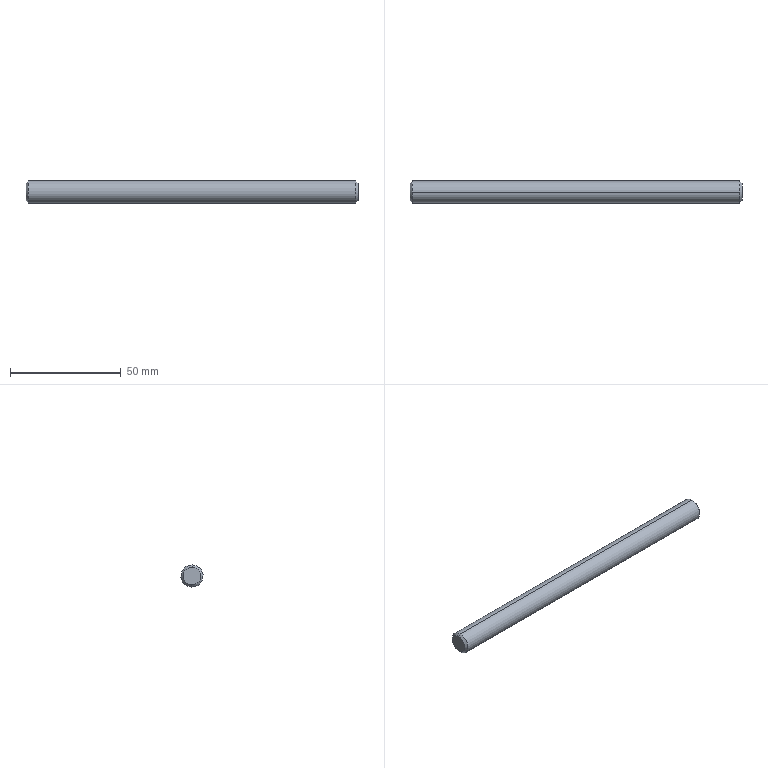Component | SolidWorks | XM-WST05-2004-1 | 1 solid | 8 faces | box 150 x 10 x 10 mm | volume 11752 mm3 | cone 4 | cylinder 2 | plane 2 | commonest cylinder face diameters 10 x2
build123d program:
from build123d import *

# Parameters (mm, degrees)
SKETCH1_R           = 5
BOSS_EXTRUDE1_DEPTH = 75
CHAMFER1_SIZE       = 1


with BuildPart() as part:
    # Sketch1 → Boss-Extrude1 (new, symmetric)
    with BuildSketch(Plane.XY):
        Circle(SKETCH1_R)
    extrude(amount=BOSS_EXTRUDE1_DEPTH, both=True)

    # Chamfer1
    chamfer1_edges = [part.edges().sort_by_distance(p)[0] for p in [
        (-5, 0, -75),
        (-5, 0, 75),
    ]]
    chamfer(chamfer1_edges, length=CHAMFER1_SIZE)


solid = part.part

# Placed as in the assembly
solid = solid.moved(Location((-160.071, 117.709, 421.25), (0, 90, 0)))
STEP:
#1=COLOUR_RGB('',0.7922,0.8196,0.9333);
#2=FILL_AREA_STYLE_COLOUR('',#1);
#3=FILL_AREA_STYLE('',(#2));
#4=SURFACE_STYLE_FILL_AREA(#3);
#5=SURFACE_SIDE_STYLE('',(#4));
#6=SURFACE_STYLE_USAGE(.BOTH.,#5);
#7=PRESENTATION_STYLE_ASSIGNMENT((#6));
#8=CARTESIAN_POINT('',(-3.349,4.637,16.427));
#9=VERTEX_POINT('',#8);
#10=CARTESIAN_POINT('',(-3.349,4.631,16.742));
#11=VERTEX_POINT('',#10);
#12=CARTESIAN_POINT('',(-3.349,4.634,16.585));
#13=DIRECTION('',(1.,0.,-0.));
#14=DIRECTION('',(0.,0.0199,-0.9998));
#15=AXIS2_PLACEMENT_3D('',#12,#13,#14);
#16=CIRCLE('',#15,0.1575);
#17=EDGE_CURVE('',#9,#11,#16,.T.);
#18=ORIENTED_EDGE('',*,*,#17,.F.);
#19=CARTESIAN_POINT('',(-3.389,4.638,16.388));
#20=VERTEX_POINT('',#19);
#21=CARTESIAN_POINT('',(-3.349,4.637,16.427));
#22=DIRECTION('',(-0.7071,0.01407,-0.707));
#23=VECTOR('',#22,39.37);
#24=LINE('',#21,#23);
#25=EDGE_CURVE('',#9,#20,#24,.T.);
#26=ORIENTED_EDGE('',*,*,#25,.T.);
#27=CARTESIAN_POINT('',(-3.389,4.63,16.781));
#28=VERTEX_POINT('',#27);
#29=CARTESIAN_POINT('',(-3.389,4.634,16.585));
#30=DIRECTION('',(-1.,-0.,0.));
#31=DIRECTION('',(0.,0.0199,-0.9998));
#32=AXIS2_PLACEMENT_3D('',#29,#30,#31);
#33=CIRCLE('',#32,0.1969);
#34=EDGE_CURVE('',#28,#20,#33,.T.);
#35=ORIENTED_EDGE('',*,*,#34,.F.);
#36=CARTESIAN_POINT('',(-3.349,4.631,16.742));
#37=DIRECTION('',(-0.7071,-0.01407,0.707));
#38=VECTOR('',#37,39.37);
#39=LINE('',#36,#38);
#40=EDGE_CURVE('',#11,#28,#39,.T.);
#41=ORIENTED_EDGE('',*,*,#40,.F.);
#42=EDGE_LOOP('',(#18,#26,#35,#41));
#43=FACE_OUTER_BOUND('',#42,.T.);
#44=CARTESIAN_POINT('',(-3.349,4.634,16.585));
#45=DIRECTION('',(-1.,-0.,0.));
#46=DIRECTION('',(0.,-0.0199,0.9998));
#47=AXIS2_PLACEMENT_3D('',#44,#45,#46);
#48=CONICAL_SURFACE('',#47,0.1575,0.7854);
#49=ADVANCED_FACE('',(#43),#48,.T.);
#50=CARTESIAN_POINT('',(-9.255,4.631,16.742));
#51=VERTEX_POINT('',#50);
#52=CARTESIAN_POINT('',(-9.255,4.637,16.427));
#53=VERTEX_POINT('',#52);
#54=CARTESIAN_POINT('',(-9.255,4.634,16.585));
#55=DIRECTION('',(-1.,-0.,0.));
#56=DIRECTION('',(0.,0.0199,-0.9998));
#57=AXIS2_PLACEMENT_3D('',#54,#55,#56);
#58=CIRCLE('',#57,0.1575);
#59=EDGE_CURVE('',#51,#53,#58,.T.);
#60=ORIENTED_EDGE('',*,*,#59,.F.);
#61=CARTESIAN_POINT('',(-9.215,4.63,16.781));
#62=VERTEX_POINT('',#61);
#63=CARTESIAN_POINT('',(-9.215,4.63,16.781));
#64=DIRECTION('',(0.7071,-0.01407,0.707));
#65=VECTOR('',#64,39.37);
#66=LINE('',#63,#65);
#67=EDGE_CURVE('',#51,#62,#66,.T.);
#68=ORIENTED_EDGE('',*,*,#67,.T.);
#69=CARTESIAN_POINT('',(-9.215,4.638,16.388));
#70=VERTEX_POINT('',#69);
#71=CARTESIAN_POINT('',(-9.215,4.634,16.585));
#72=DIRECTION('',(1.,0.,-0.));
#73=DIRECTION('',(0.,0.0199,-0.9998));
#74=AXIS2_PLACEMENT_3D('',#71,#72,#73);
#75=CIRCLE('',#74,0.1969);
#76=EDGE_CURVE('',#70,#62,#75,.T.);
#77=ORIENTED_EDGE('',*,*,#76,.F.);
#78=CARTESIAN_POINT('',(-9.215,4.638,16.388));
#79=DIRECTION('',(0.7071,0.01407,-0.707));
#80=VECTOR('',#79,39.37);
#81=LINE('',#78,#80);
#82=EDGE_CURVE('',#53,#70,#81,.T.);
#83=ORIENTED_EDGE('',*,*,#82,.F.);
#84=EDGE_LOOP('',(#60,#68,#77,#83));
#85=FACE_OUTER_BOUND('',#84,.T.);
#86=CARTESIAN_POINT('',(-9.215,4.634,16.585));
#87=DIRECTION('',(1.,0.,-0.));
#88=DIRECTION('',(0.,0.0199,-0.9998));
#89=AXIS2_PLACEMENT_3D('',#86,#87,#88);
#90=CONICAL_SURFACE('',#89,0.1969,0.7854);
#91=ADVANCED_FACE('',(#85),#90,.T.);
#92=ORIENTED_EDGE('',*,*,#34,.T.);
#93=CARTESIAN_POINT('',(-3.349,4.638,16.388));
#94=DIRECTION('',(-1.,-0.,0.));
#95=VECTOR('',#94,39.37);
#96=LINE('',#93,#95);
#97=EDGE_CURVE('',#20,#70,#96,.T.);
#98=ORIENTED_EDGE('',*,*,#97,.T.);
#99=ORIENTED_EDGE('',*,*,#76,.T.);
#100=CARTESIAN_POINT('',(-3.349,4.63,16.781));
#101=DIRECTION('',(-1.,-0.,0.));
#102=VECTOR('',#101,39.37);
#103=LINE('',#100,#102);
#104=EDGE_CURVE('',#28,#62,#103,.T.);
#105=ORIENTED_EDGE('',*,*,#104,.F.);
#106=EDGE_LOOP('',(#92,#98,#99,#105));
#107=FACE_OUTER_BOUND('',#106,.T.);
#108=CARTESIAN_POINT('',(-3.349,4.634,16.585));
#109=DIRECTION('',(-1.,-0.,0.));
#110=DIRECTION('',(0.,-0.0199,0.9998));
#111=AXIS2_PLACEMENT_3D('',#108,#109,#110);
#112=CYLINDRICAL_SURFACE('',#111,0.1969);
#113=ADVANCED_FACE('',(#107),#112,.T.);
#114=ORIENTED_EDGE('',*,*,#97,.F.);
#115=CARTESIAN_POINT('',(-3.389,4.634,16.585));
#116=DIRECTION('',(-1.,-0.,0.));
#117=DIRECTION('',(0.,0.0199,-0.9998));
#118=AXIS2_PLACEMENT_3D('',#115,#116,#117);
#119=CIRCLE('',#118,0.1969);
#120=EDGE_CURVE('',#20,#28,#119,.T.);
#121=ORIENTED_EDGE('',*,*,#120,.T.);
#122=ORIENTED_EDGE('',*,*,#104,.T.);
#123=CARTESIAN_POINT('',(-9.215,4.634,16.585));
#124=DIRECTION('',(1.,0.,-0.));
#125=DIRECTION('',(0.,0.0199,-0.9998));
#126=AXIS2_PLACEMENT_3D('',#123,#124,#125);
#127=CIRCLE('',#126,0.1969);
#128=EDGE_CURVE('',#62,#70,#127,.T.);
#129=ORIENTED_EDGE('',*,*,#128,.T.);
#130=EDGE_LOOP('',(#114,#121,#122,#129));
#131=FACE_OUTER_BOUND('',#130,.T.);
#132=CARTESIAN_POINT('',(-3.349,4.634,16.585));
#133=DIRECTION('',(-1.,-0.,0.));
#134=DIRECTION('',(0.,-0.0199,0.9998));
#135=AXIS2_PLACEMENT_3D('',#132,#133,#134);
#136=CYLINDRICAL_SURFACE('',#135,0.1969);
#137=ADVANCED_FACE('',(#131),#136,.T.);
#138=CARTESIAN_POINT('',(-3.349,4.634,16.585));
#139=DIRECTION('',(1.,0.,-0.));
#140=DIRECTION('',(0.,0.0199,-0.9998));
#141=AXIS2_PLACEMENT_3D('',#138,#139,#140);
#142=CIRCLE('',#141,0.1575);
#143=EDGE_CURVE('',#11,#9,#142,.T.);
#144=ORIENTED_EDGE('',*,*,#143,.T.);
#145=ORIENTED_EDGE('',*,*,#17,.T.);
#146=EDGE_LOOP('',(#144,#145));
#147=FACE_OUTER_BOUND('',#146,.T.);
#148=CARTESIAN_POINT('',(-3.349,4.634,16.585));
#149=DIRECTION('',(1.,0.,-0.));
#150=DIRECTION('',(-0.,0.0199,-0.9998));
#151=AXIS2_PLACEMENT_3D('',#148,#149,#150);
#152=PLANE('',#151);
#153=ADVANCED_FACE('',(#147),#152,.T.);
#154=CARTESIAN_POINT('',(-9.255,4.634,16.585));
#155=DIRECTION('',(-1.,-0.,0.));
#156=DIRECTION('',(0.,0.0199,-0.9998));
#157=AXIS2_PLACEMENT_3D('',#154,#155,#156);
#158=CIRCLE('',#157,0.1575);
#159=EDGE_CURVE('',#53,#51,#158,.T.);
#160=ORIENTED_EDGE('',*,*,#159,.T.);
#161=ORIENTED_EDGE('',*,*,#59,.T.);
#162=EDGE_LOOP('',(#160,#161));
#163=FACE_OUTER_BOUND('',#162,.T.);
#164=CARTESIAN_POINT('',(-9.255,4.634,16.585));
#165=DIRECTION('',(1.,0.,-0.));
#166=DIRECTION('',(-0.,0.0199,-0.9998));
#167=AXIS2_PLACEMENT_3D('',#164,#165,#166);
#168=PLANE('',#167);
#169=ADVANCED_FACE('',(#163),#168,.F.);
#170=ORIENTED_EDGE('',*,*,#67,.F.);
#171=ORIENTED_EDGE('',*,*,#159,.F.);
#172=ORIENTED_EDGE('',*,*,#82,.T.);
#173=ORIENTED_EDGE('',*,*,#128,.F.);
#174=EDGE_LOOP('',(#170,#171,#172,#173));
#175=FACE_OUTER_BOUND('',#174,.T.);
#176=CARTESIAN_POINT('',(-9.215,4.634,16.585));
#177=DIRECTION('',(1.,0.,-0.));
#178=DIRECTION('',(0.,0.0199,-0.9998));
#179=AXIS2_PLACEMENT_3D('',#176,#177,#178);
#180=CONICAL_SURFACE('',#179,0.1969,0.7854);
#181=ADVANCED_FACE('',(#175),#180,.T.);
#182=ORIENTED_EDGE('',*,*,#25,.F.);
#183=ORIENTED_EDGE('',*,*,#143,.F.);
#184=ORIENTED_EDGE('',*,*,#40,.T.);
#185=ORIENTED_EDGE('',*,*,#120,.F.);
#186=EDGE_LOOP('',(#182,#183,#184,#185));
#187=FACE_OUTER_BOUND('',#186,.T.);
#188=CARTESIAN_POINT('',(-3.349,4.634,16.585));
#189=DIRECTION('',(-1.,-0.,0.));
#190=DIRECTION('',(0.,-0.0199,0.9998));
#191=AXIS2_PLACEMENT_3D('',#188,#189,#190);
#192=CONICAL_SURFACE('',#191,0.1575,0.7854);
#193=ADVANCED_FACE('',(#187),#192,.T.);
#194=CLOSED_SHELL('',(#49,#91,#113,#137,#153,#169,#181,#193));
#195=MANIFOLD_SOLID_BREP('',#194);
#196=STYLED_ITEM('',(#7),#195);
#197=PRESENTATION_LAYER_ASSIGNMENT('','',(#196));
#198=(LENGTH_UNIT()NAMED_UNIT(*)SI_UNIT($,.METRE.));
#199=LENGTH_MEASURE_WITH_UNIT(LENGTH_MEASURE(0.0254),#198);
#200=DIMENSIONAL_EXPONENTS(1.,0.,0.,0.,0.,0.,0.);
#201=(CONVERSION_BASED_UNIT('',#199)LENGTH_UNIT()NAMED_UNIT(#200));
#202=UNCERTAINTY_MEASURE_WITH_UNIT(LENGTH_MEASURE(0.00001),#201,'','');
#203=(NAMED_UNIT(*)PLANE_ANGLE_UNIT()SI_UNIT($,.RADIAN.));
#204=(NAMED_UNIT(*)SI_UNIT($,.STERADIAN.)SOLID_ANGLE_UNIT());
#205=(GEOMETRIC_REPRESENTATION_CONTEXT(3)GLOBAL_UNCERTAINTY_ASSIGNED_CONTEXT((#202))GLOBAL_UNIT_ASSIGNED_CONTEXT((#201,#203,#204))REPRESENTATION_CONTEXT('',''));
#206=MECHANICAL_DESIGN_GEOMETRIC_PRESENTATION_REPRESENTATION('',(#196),#205);
#207=CARTESIAN_POINT('',(0.,0.,0.));
#208=DIRECTION('',(0.,0.,1.));
#209=DIRECTION('',(1.,0.,0.));
#210=AXIS2_PLACEMENT_3D('',#207,#208,#209);
#211=(LENGTH_UNIT()NAMED_UNIT(*)SI_UNIT($,.METRE.));
#212=LENGTH_MEASURE_WITH_UNIT(LENGTH_MEASURE(0.0254),#211);
#213=DIMENSIONAL_EXPONENTS(1.,0.,0.,0.,0.,0.,0.);
#214=(CONVERSION_BASED_UNIT('',#212)LENGTH_UNIT()NAMED_UNIT(#213));
#215=UNCERTAINTY_MEASURE_WITH_UNIT(LENGTH_MEASURE(0.00001),#214,'','');
#216=(NAMED_UNIT(*)PLANE_ANGLE_UNIT()SI_UNIT($,.RADIAN.));
#217=(NAMED_UNIT(*)SI_UNIT($,.STERADIAN.)SOLID_ANGLE_UNIT());
#218=(GEOMETRIC_REPRESENTATION_CONTEXT(3)GLOBAL_UNCERTAINTY_ASSIGNED_CONTEXT((#215))GLOBAL_UNIT_ASSIGNED_CONTEXT((#214,#216,#217))REPRESENTATION_CONTEXT('',''));
#219=ADVANCED_BREP_SHAPE_REPRESENTATION('',(#195,#210),#218);